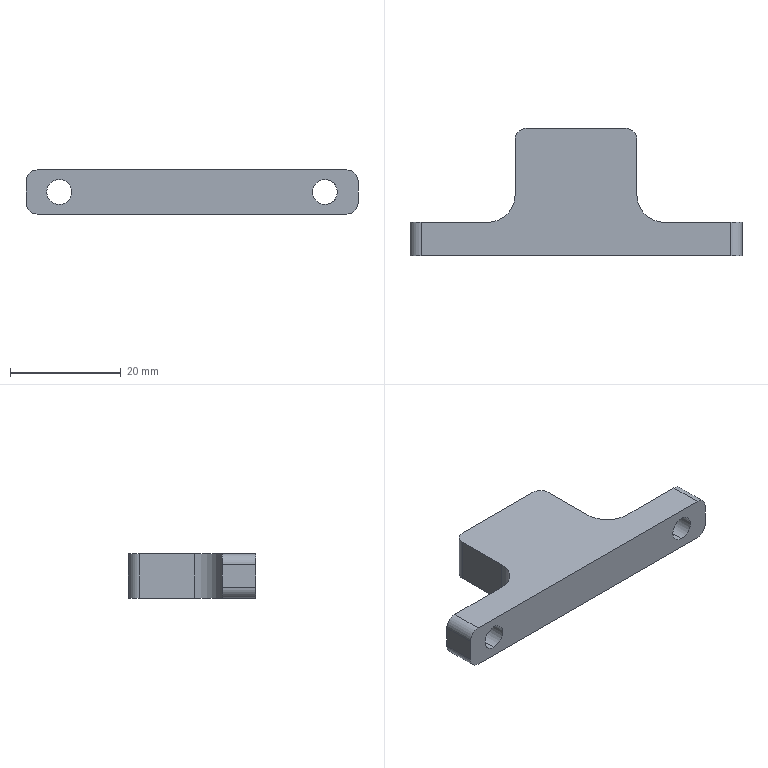CAM job | Mastercam | mm | 10 operations | part box 60 x 23 x 8
1. Facing | 24 - 100 平铣刀
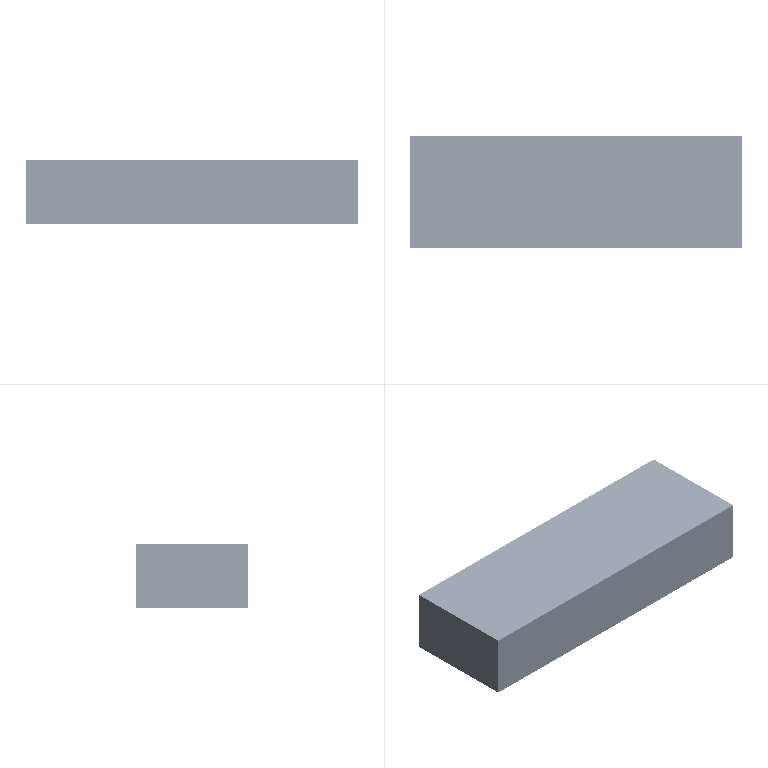2. 3D High Speed (Dynamic OptiRough) | 12 - 12 平铣刀
3. Contour (2D) | 12 - 12 平铣刀
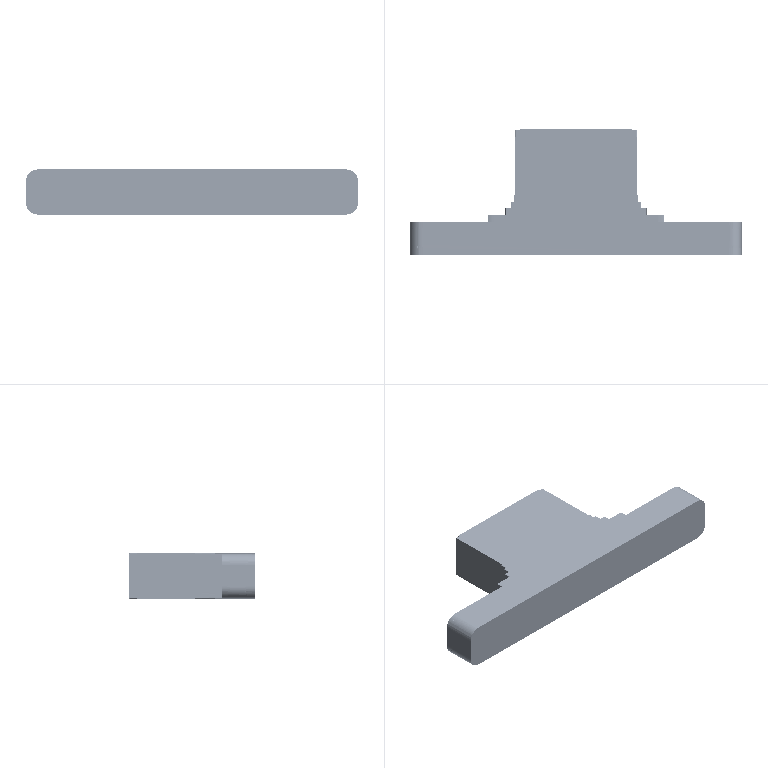4. Contour (2D) | 12 - 12 平铣刀
5. Contour (2D) | 12 - 12 平铣刀
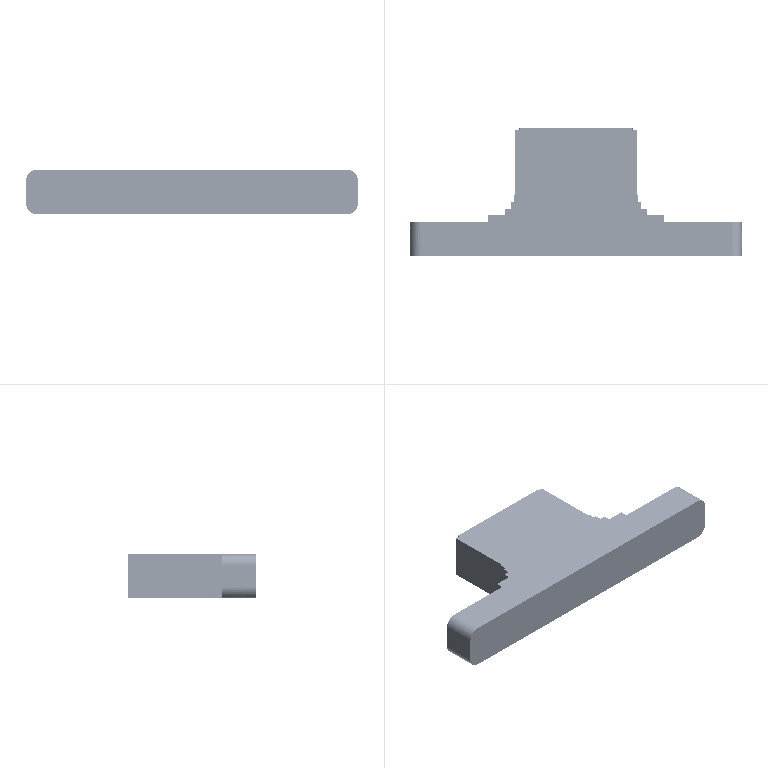6. Surface Finish Flowline | 9 - 8 圆鼻铣刀
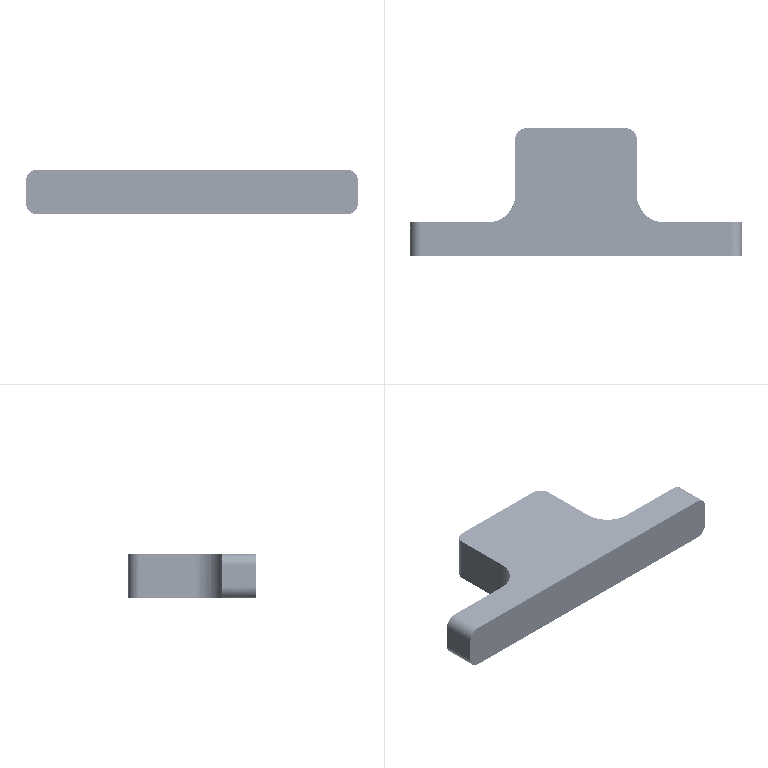7. Drill/Counterbore | 7 - 4 倒角刀
8. Deburr 5-axis | 5 - 4 球刀/圆鼻铣刀
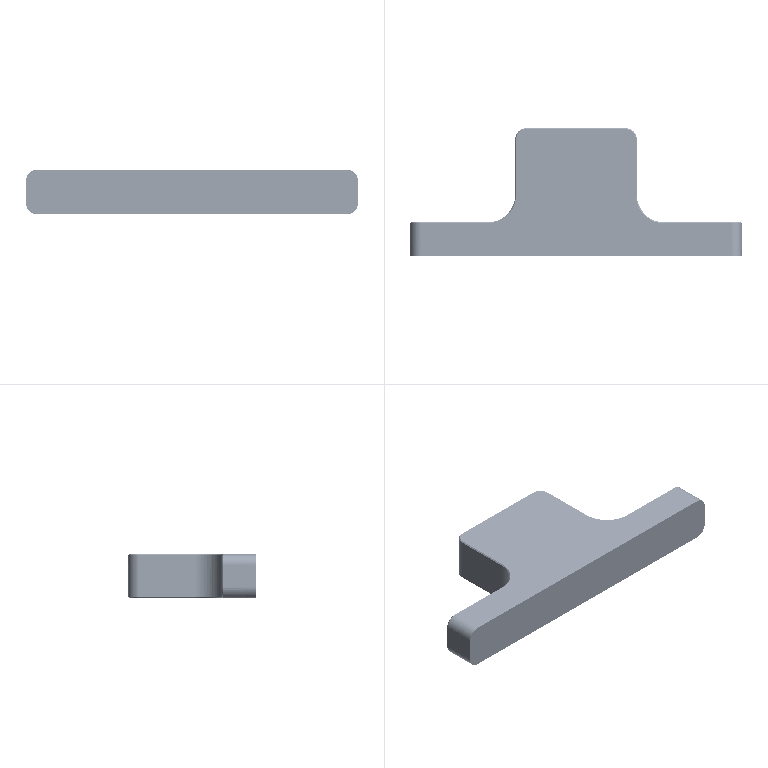9. Facing | 24 - 100 平铣刀
10. Contour (2D chamfer) | 7 - 4 倒角刀